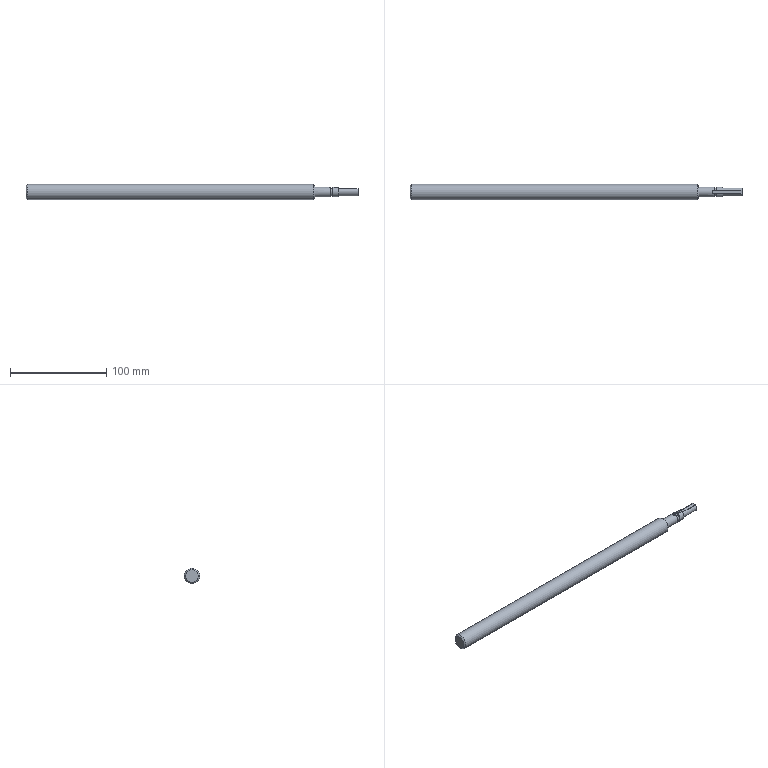Component | NX | SLIDE_SCREW | 1 solid | 17 faces | volume 62976 mm3 | plane 9 | cylinder 6 | cone 2 | commonest cylinder face diameters 10 x2 8 x2 3.5 x1 16 x1